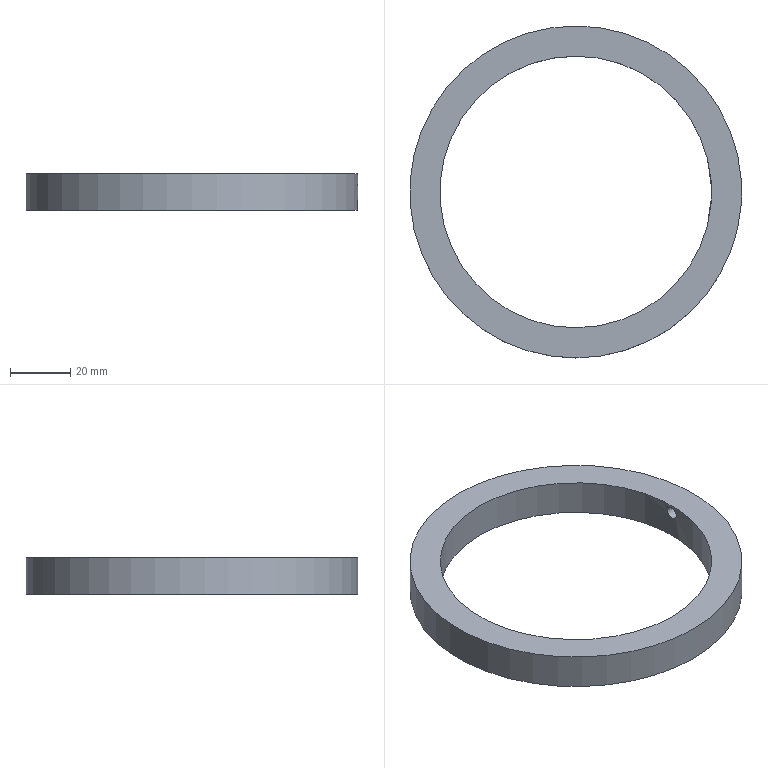Component | NX | CA6140-ZHUZHOU-ZHOUTAO4 | 1 solid | 5 faces | box 110 x 110 x 12 mm | volume 37574 mm3 | cylinder 3 | plane 2 | commonest cylinder face diameters 110 x1 90 x1 4 x1
STEP:
#1=CARTESIAN_POINT('',(0.,0.,0.));
#2=DIRECTION('',(0.,0.,1.));
#3=DIRECTION('',(1.,0.,0.));
#4=AXIS2_PLACEMENT_3D('',#1,#2,#3);
#5=CARTESIAN_POINT('',(0.03562,-45.,-99.951));
#6=VERTEX_POINT('',#5);
#7=CARTESIAN_POINT('',(-0.,-0.,-99.951));
#8=DIRECTION('',(0.,0.,1.));
#9=DIRECTION('',(0.0007915,-1.,0.));
#10=AXIS2_PLACEMENT_3D('',#7,#8,#9);
#11=CIRCLE('',#10,45.);
#12=CARTESIAN_POINT('',(-0.,-0.,-99.951));
#13=DIRECTION('',(0.,0.,-1.));
#14=DIRECTION('',(-0.0007915,1.,0.));
#15=AXIS2_PLACEMENT_3D('',#12,#13,#14);
#16=PLANE('',#15);
#17=CARTESIAN_POINT('',(-45.,0.));
#18=CARTESIAN_POINT('',(-45.,77.942));
#19=CARTESIAN_POINT('',(22.5,38.971));
#20=CARTESIAN_POINT('',(90.,0.));
#21=CARTESIAN_POINT('',(22.5,-38.971));
#22=CARTESIAN_POINT('',(-45.,-77.942));
#23=CARTESIAN_POINT('',(-45.,0.));
#24=(BOUNDED_CURVE()B_SPLINE_CURVE(2,(#17,#18,#19,#20,#21,#22,#23),.UNSPECIFIED.,.T.,.F.)B_SPLINE_CURVE_WITH_KNOTS((1,2,2,2,2,1),(-2.094,0.,2.094,4.189,6.283,8.378),.UNSPECIFIED.)CURVE()GEOMETRIC_REPRESENTATION_ITEM()RATIONAL_B_SPLINE_CURVE((1.,0.5,1.,0.5,1.,0.5,1.))REPRESENTATION_ITEM(''));
#25=(GEOMETRIC_REPRESENTATION_CONTEXT(2)PARAMETRIC_REPRESENTATION_CONTEXT()REPRESENTATION_CONTEXT('',''));
#26=DEFINITIONAL_REPRESENTATION('',(#24),#25);
#27=PCURVE('',#16,#26);
#28=CARTESIAN_POINT('',(-0.,-0.,-99.951));
#29=DIRECTION('',(0.,0.,1.));
#30=DIRECTION('',(0.0007915,-1.,0.));
#31=AXIS2_PLACEMENT_3D('',#28,#29,#30);
#32=CYLINDRICAL_SURFACE('',#31,45.);
#33=CARTESIAN_POINT('',(0.,0.));
#34=DIRECTION('',(1.,0.));
#35=VECTOR('',#34,1.);
#36=LINE('',#33,#35);
#37=(GEOMETRIC_REPRESENTATION_CONTEXT(2)PARAMETRIC_REPRESENTATION_CONTEXT()REPRESENTATION_CONTEXT('',''));
#38=DEFINITIONAL_REPRESENTATION('',(#36),#37);
#39=PCURVE('',#32,#38);
#40=SURFACE_CURVE('',#11,(#27,#39),.PCURVE_S1.);
#41=EDGE_CURVE('',#6,#6,#40,.T.);
#42=ORIENTED_EDGE('',*,*,#41,.T.);
#43=EDGE_LOOP('',(#42));
#44=FACE_BOUND('',#43,.T.);
#45=CARTESIAN_POINT('',(0.04353,-55.,-99.951));
#46=VERTEX_POINT('',#45);
#47=CARTESIAN_POINT('',(-0.04353,55.,-99.951));
#48=VERTEX_POINT('',#47);
#49=CARTESIAN_POINT('',(-0.,-0.,-99.951));
#50=DIRECTION('',(0.,0.,1.));
#51=DIRECTION('',(0.0007915,-1.,0.));
#52=AXIS2_PLACEMENT_3D('',#49,#50,#51);
#53=CIRCLE('',#52,55.);
#54=CARTESIAN_POINT('',(-55.,0.));
#55=CARTESIAN_POINT('',(-55.,95.263));
#56=CARTESIAN_POINT('',(27.5,47.631));
#57=CARTESIAN_POINT('',(110.,0.));
#58=CARTESIAN_POINT('',(27.5,-47.631));
#59=CARTESIAN_POINT('',(-55.,-95.263));
#60=CARTESIAN_POINT('',(-55.,0.));
#61=(BOUNDED_CURVE()B_SPLINE_CURVE(2,(#54,#55,#56,#57,#58,#59,#60),.UNSPECIFIED.,.T.,.F.)B_SPLINE_CURVE_WITH_KNOTS((1,2,2,2,2,1),(-2.094,0.,2.094,4.189,6.283,8.378),.UNSPECIFIED.)CURVE()GEOMETRIC_REPRESENTATION_ITEM()RATIONAL_B_SPLINE_CURVE((1.,0.5,1.,0.5,1.,0.5,1.))REPRESENTATION_ITEM(''));
#62=(GEOMETRIC_REPRESENTATION_CONTEXT(2)PARAMETRIC_REPRESENTATION_CONTEXT()REPRESENTATION_CONTEXT('',''));
#63=DEFINITIONAL_REPRESENTATION('',(#61),#62);
#64=PCURVE('',#16,#63);
#65=CARTESIAN_POINT('',(-0.,-0.,-87.951));
#66=DIRECTION('',(0.,0.,-1.));
#67=DIRECTION('',(-0.0007915,1.,0.));
#68=AXIS2_PLACEMENT_3D('',#65,#66,#67);
#69=CYLINDRICAL_SURFACE('',#68,55.);
#70=CARTESIAN_POINT('',(3.142,12.));
#71=DIRECTION('',(-1.,0.));
#72=VECTOR('',#71,1.);
#73=LINE('',#70,#72);
#74=(GEOMETRIC_REPRESENTATION_CONTEXT(2)PARAMETRIC_REPRESENTATION_CONTEXT()REPRESENTATION_CONTEXT('',''));
#75=DEFINITIONAL_REPRESENTATION('',(#73),#74);
#76=PCURVE('',#69,#75);
#77=SURFACE_CURVE('',#53,(#64,#76),.PCURVE_S1.);
#78=EDGE_CURVE('',#46,#48,#77,.T.);
#79=ORIENTED_EDGE('',*,*,#78,.F.);
#80=CARTESIAN_POINT('',(-0.,-0.,-99.951));
#81=DIRECTION('',(0.,0.,1.));
#82=DIRECTION('',(0.0007915,-1.,0.));
#83=AXIS2_PLACEMENT_3D('',#80,#81,#82);
#84=CIRCLE('',#83,55.);
#85=CARTESIAN_POINT('',(-55.,0.));
#86=CARTESIAN_POINT('',(-55.,95.263));
#87=CARTESIAN_POINT('',(27.5,47.631));
#88=CARTESIAN_POINT('',(110.,0.));
#89=CARTESIAN_POINT('',(27.5,-47.631));
#90=CARTESIAN_POINT('',(-55.,-95.263));
#91=CARTESIAN_POINT('',(-55.,0.));
#92=(BOUNDED_CURVE()B_SPLINE_CURVE(2,(#85,#86,#87,#88,#89,#90,#91),.UNSPECIFIED.,.T.,.F.)B_SPLINE_CURVE_WITH_KNOTS((1,2,2,2,2,1),(-2.094,0.,2.094,4.189,6.283,8.378),.UNSPECIFIED.)CURVE()GEOMETRIC_REPRESENTATION_ITEM()RATIONAL_B_SPLINE_CURVE((1.,0.5,1.,0.5,1.,0.5,1.))REPRESENTATION_ITEM(''));
#93=(GEOMETRIC_REPRESENTATION_CONTEXT(2)PARAMETRIC_REPRESENTATION_CONTEXT()REPRESENTATION_CONTEXT('',''));
#94=DEFINITIONAL_REPRESENTATION('',(#92),#93);
#95=PCURVE('',#16,#94);
#96=CARTESIAN_POINT('',(9.425,12.));
#97=DIRECTION('',(-1.,0.));
#98=VECTOR('',#97,1.);
#99=LINE('',#96,#98);
#100=(GEOMETRIC_REPRESENTATION_CONTEXT(2)PARAMETRIC_REPRESENTATION_CONTEXT()REPRESENTATION_CONTEXT('',''));
#101=DEFINITIONAL_REPRESENTATION('',(#99),#100);
#102=PCURVE('',#69,#101);
#103=SURFACE_CURVE('',#84,(#95,#102),.PCURVE_S1.);
#104=EDGE_CURVE('',#48,#46,#103,.T.);
#105=ORIENTED_EDGE('',*,*,#104,.F.);
#106=EDGE_LOOP('',(#79,#105));
#107=FACE_BOUND('',#106,.T.);
#108=ADVANCED_FACE('',(#44,#107),#16,.T.);
#109=CARTESIAN_POINT('',(0.03562,-45.,-87.951));
#110=VERTEX_POINT('',#109);
#111=CARTESIAN_POINT('',(-0.,-0.,-87.951));
#112=DIRECTION('',(0.,0.,1.));
#113=DIRECTION('',(0.0007915,-1.,0.));
#114=AXIS2_PLACEMENT_3D('',#111,#112,#113);
#115=CIRCLE('',#114,45.);
#116=CARTESIAN_POINT('',(-0.,-0.,-87.951));
#117=DIRECTION('',(0.,0.,1.));
#118=DIRECTION('',(0.0007915,-1.,0.));
#119=AXIS2_PLACEMENT_3D('',#116,#117,#118);
#120=PLANE('',#119);
#121=CARTESIAN_POINT('',(0.,0.));
#122=DIRECTION('',(1.,0.));
#123=AXIS2_PLACEMENT_2D('',#121,#122);
#124=CIRCLE('',#123,45.);
#125=(GEOMETRIC_REPRESENTATION_CONTEXT(2)PARAMETRIC_REPRESENTATION_CONTEXT()REPRESENTATION_CONTEXT('',''));
#126=DEFINITIONAL_REPRESENTATION('',(#124),#125);
#127=PCURVE('',#120,#126);
#128=CARTESIAN_POINT('',(0.,12.));
#129=DIRECTION('',(1.,0.));
#130=VECTOR('',#129,1.);
#131=LINE('',#128,#130);
#132=(GEOMETRIC_REPRESENTATION_CONTEXT(2)PARAMETRIC_REPRESENTATION_CONTEXT()REPRESENTATION_CONTEXT('',''));
#133=DEFINITIONAL_REPRESENTATION('',(#131),#132);
#134=PCURVE('',#32,#133);
#135=SURFACE_CURVE('',#115,(#127,#134),.PCURVE_S1.);
#136=EDGE_CURVE('',#110,#110,#135,.T.);
#137=ORIENTED_EDGE('',*,*,#136,.F.);
#138=EDGE_LOOP('',(#137));
#139=FACE_BOUND('',#138,.T.);
#140=CARTESIAN_POINT('',(-0.04353,55.,-87.951));
#141=VERTEX_POINT('',#140);
#142=CARTESIAN_POINT('',(-0.,-0.,-87.951));
#143=DIRECTION('',(0.,0.,-1.));
#144=DIRECTION('',(-0.0007915,1.,0.));
#145=AXIS2_PLACEMENT_3D('',#142,#143,#144);
#146=CIRCLE('',#145,55.);
#147=CARTESIAN_POINT('',(-55.,0.));
#148=CARTESIAN_POINT('',(-55.,95.263));
#149=CARTESIAN_POINT('',(27.5,47.631));
#150=CARTESIAN_POINT('',(110.,0.));
#151=CARTESIAN_POINT('',(27.5,-47.631));
#152=CARTESIAN_POINT('',(-55.,-95.263));
#153=CARTESIAN_POINT('',(-55.,0.));
#154=(BOUNDED_CURVE()B_SPLINE_CURVE(2,(#147,#148,#149,#150,#151,#152,#153),.UNSPECIFIED.,.T.,.F.)B_SPLINE_CURVE_WITH_KNOTS((1,2,2,2,2,1),(-2.094,0.,2.094,4.189,6.283,8.378),.UNSPECIFIED.)CURVE()GEOMETRIC_REPRESENTATION_ITEM()RATIONAL_B_SPLINE_CURVE((1.,0.5,1.,0.5,1.,0.5,1.))REPRESENTATION_ITEM(''));
#155=(GEOMETRIC_REPRESENTATION_CONTEXT(2)PARAMETRIC_REPRESENTATION_CONTEXT()REPRESENTATION_CONTEXT('',''));
#156=DEFINITIONAL_REPRESENTATION('',(#154),#155);
#157=PCURVE('',#120,#156);
#158=CARTESIAN_POINT('',(0.,0.));
#159=DIRECTION('',(1.,0.));
#160=VECTOR('',#159,1.);
#161=LINE('',#158,#160);
#162=(GEOMETRIC_REPRESENTATION_CONTEXT(2)PARAMETRIC_REPRESENTATION_CONTEXT()REPRESENTATION_CONTEXT('',''));
#163=DEFINITIONAL_REPRESENTATION('',(#161),#162);
#164=PCURVE('',#69,#163);
#165=SURFACE_CURVE('',#146,(#157,#164),.PCURVE_S1.);
#166=EDGE_CURVE('',#141,#141,#165,.T.);
#167=ORIENTED_EDGE('',*,*,#166,.F.);
#168=EDGE_LOOP('',(#167));
#169=FACE_BOUND('',#168,.T.);
#170=ADVANCED_FACE('',(#139,#169),#120,.T.);
#171=ORIENTED_EDGE('',*,*,#78,.T.);
#172=CARTESIAN_POINT('',(-0.04353,55.,-87.951));
#173=CARTESIAN_POINT('',(-0.04353,55.,-99.951));
#174=B_SPLINE_CURVE_WITH_KNOTS('',1,(#172,#173),.UNSPECIFIED.,.F.,.F.,(2,2),(0.,12.),.PIECEWISE_BEZIER_KNOTS.);
#175=CARTESIAN_POINT('',(0.,0.));
#176=DIRECTION('',(0.,1.));
#177=VECTOR('',#176,1.);
#178=LINE('',#175,#177);
#179=(GEOMETRIC_REPRESENTATION_CONTEXT(2)PARAMETRIC_REPRESENTATION_CONTEXT()REPRESENTATION_CONTEXT('',''));
#180=DEFINITIONAL_REPRESENTATION('',(#178),#179);
#181=PCURVE('',#69,#180);
#182=CARTESIAN_POINT('',(6.283,0.));
#183=DIRECTION('',(0.,1.));
#184=VECTOR('',#183,1.);
#185=LINE('',#182,#184);
#186=(GEOMETRIC_REPRESENTATION_CONTEXT(2)PARAMETRIC_REPRESENTATION_CONTEXT()REPRESENTATION_CONTEXT('',''));
#187=DEFINITIONAL_REPRESENTATION('',(#185),#186);
#188=PCURVE('',#69,#187);
#189=SEAM_CURVE('',#174,(#181,#188),.PCURVE_S1.);
#190=EDGE_CURVE('',#141,#48,#189,.T.);
#191=ORIENTED_EDGE('',*,*,#190,.F.);
#192=ORIENTED_EDGE('',*,*,#166,.T.);
#193=ORIENTED_EDGE('',*,*,#190,.T.);
#194=ORIENTED_EDGE('',*,*,#104,.T.);
#195=EDGE_LOOP('',(#171,#191,#192,#193,#194));
#196=FACE_BOUND('',#195,.T.);
#197=CARTESIAN_POINT('',(55.,0.04365,-88.951));
#198=VERTEX_POINT('',#197);
#199=CARTESIAN_POINT('',(55.,0.04365,-88.951));
#200=CARTESIAN_POINT('',(55.,-0.1801,-88.951));
#201=CARTESIAN_POINT('',(54.999,-0.407,-88.989));
#202=CARTESIAN_POINT('',(54.997,-0.6181,-89.063));
#203=CARTESIAN_POINT('',(54.994,-0.8293,-89.137));
#204=CARTESIAN_POINT('',(54.991,-1.031,-89.249));
#205=CARTESIAN_POINT('',(54.987,-1.205,-89.389));
#206=CARTESIAN_POINT('',(54.983,-1.38,-89.528));
#207=CARTESIAN_POINT('',(54.979,-1.533,-89.7));
#208=CARTESIAN_POINT('',(54.975,-1.652,-89.89));
#209=CARTESIAN_POINT('',(54.972,-1.771,-90.08));
#210=CARTESIAN_POINT('',(54.969,-1.858,-90.293));
#211=CARTESIAN_POINT('',(54.967,-1.907,-90.511));
#212=CARTESIAN_POINT('',(54.965,-1.957,-90.729));
#213=CARTESIAN_POINT('',(54.965,-1.969,-90.959));
#214=CARTESIAN_POINT('',(54.966,-1.943,-91.182));
#215=CARTESIAN_POINT('',(54.967,-1.917,-91.404));
#216=CARTESIAN_POINT('',(54.969,-1.853,-91.625));
#217=CARTESIAN_POINT('',(54.972,-1.755,-91.826));
#218=CARTESIAN_POINT('',(54.975,-1.657,-92.027));
#219=CARTESIAN_POINT('',(54.979,-1.523,-92.214));
#220=CARTESIAN_POINT('',(54.983,-1.364,-92.371));
#221=CARTESIAN_POINT('',(54.987,-1.205,-92.529));
#222=CARTESIAN_POINT('',(54.991,-1.017,-92.661));
#223=CARTESIAN_POINT('',(54.994,-0.8143,-92.757));
#224=CARTESIAN_POINT('',(54.997,-0.612,-92.853));
#225=CARTESIAN_POINT('',(54.999,-0.3904,-92.916));
#226=CARTESIAN_POINT('',(55.,-0.1678,-92.939));
#227=CARTESIAN_POINT('',(55.,0.05473,-92.963));
#228=CARTESIAN_POINT('',(55.,0.2844,-92.949));
#229=CARTESIAN_POINT('',(54.998,0.5022,-92.897));
#230=CARTESIAN_POINT('',(54.996,0.7199,-92.846));
#231=CARTESIAN_POINT('',(54.992,0.9318,-92.757));
#232=CARTESIAN_POINT('',(54.989,1.12,-92.636));
#233=CARTESIAN_POINT('',(54.985,1.309,-92.516));
#234=CARTESIAN_POINT('',(54.98,1.479,-92.361));
#235=CARTESIAN_POINT('',(54.976,1.617,-92.185));
#236=CARTESIAN_POINT('',(54.972,1.756,-92.009));
#237=CARTESIAN_POINT('',(54.968,1.865,-91.806));
#238=CARTESIAN_POINT('',(54.966,1.937,-91.594));
#239=CARTESIAN_POINT('',(54.963,2.009,-91.382));
#240=CARTESIAN_POINT('',(54.962,2.046,-91.155));
#241=CARTESIAN_POINT('',(54.962,2.044,-90.931));
#242=CARTESIAN_POINT('',(54.962,2.041,-90.707));
#243=CARTESIAN_POINT('',(54.964,2.001,-90.481));
#244=CARTESIAN_POINT('',(54.966,1.924,-90.271));
#245=CARTESIAN_POINT('',(54.969,1.848,-90.06));
#246=CARTESIAN_POINT('',(54.973,1.735,-89.86));
#247=CARTESIAN_POINT('',(54.977,1.594,-89.687));
#248=CARTESIAN_POINT('',(54.981,1.452,-89.513));
#249=CARTESIAN_POINT('',(54.985,1.279,-89.362));
#250=CARTESIAN_POINT('',(54.989,1.088,-89.245));
#251=CARTESIAN_POINT('',(54.993,0.8971,-89.128));
#252=CARTESIAN_POINT('',(54.996,0.6833,-89.043));
#253=CARTESIAN_POINT('',(54.998,0.4644,-88.995));
#254=CARTESIAN_POINT('',(54.999,0.3265,-88.966));
#255=CARTESIAN_POINT('',(55.,0.1847,-88.951));
#256=CARTESIAN_POINT('',(55.,0.04365,-88.951));
#257=B_SPLINE_CURVE_WITH_KNOTS('',3,(#199,#200,#201,#202,#203,#204,#205,#206,#207,#208,#209,#210,#211,#212,#213,#214,#215,#216,#217,#218,#219,#220,#221,#222,#223,#224,#225,#226,#227,#228,#229,#230,#231,#232,#233,#234,#235,#236,#237,#238,#239,#240,#241,#242,#243,#244,#245,#246,#247,#248,#249,#250,#251,#252,#253,#254,#255,#256),.UNSPECIFIED.,.T.,.F.,(1,3,3,3,3,3,3,3,3,3,3,3,3,3,3,3,3,3,3,3,3,1),(-0.03354,0.,0.05368,0.1074,0.1611,0.2148,0.2685,0.3221,0.3758,0.4295,0.4832,0.5369,0.5906,0.6443,0.698,0.7517,0.8054,0.859,0.9127,0.9665,1.,1.054),.UNSPECIFIED.);
#258=CARTESIAN_POINT('',(1.571,0.9999));
#259=CARTESIAN_POINT('',(1.572,0.9999));
#260=CARTESIAN_POINT('',(1.573,1.003));
#261=CARTESIAN_POINT('',(1.576,1.019));
#262=CARTESIAN_POINT('',(1.579,1.044));
#263=CARTESIAN_POINT('',(1.581,1.079));
#264=CARTESIAN_POINT('',(1.584,1.124));
#265=CARTESIAN_POINT('',(1.586,1.179));
#266=CARTESIAN_POINT('',(1.588,1.243));
#267=CARTESIAN_POINT('',(1.59,1.316));
#268=CARTESIAN_POINT('',(1.593,1.398));
#269=CARTESIAN_POINT('',(1.595,1.487));
#270=CARTESIAN_POINT('',(1.597,1.584));
#271=CARTESIAN_POINT('',(1.598,1.689));
#272=CARTESIAN_POINT('',(1.6,1.8));
#273=CARTESIAN_POINT('',(1.601,1.917));
#274=CARTESIAN_POINT('',(1.603,2.04));
#275=CARTESIAN_POINT('',(1.604,2.168));
#276=CARTESIAN_POINT('',(1.605,2.3));
#277=CARTESIAN_POINT('',(1.606,2.436));
#278=CARTESIAN_POINT('',(1.606,2.574));
#279=CARTESIAN_POINT('',(1.607,2.714));
#280=CARTESIAN_POINT('',(1.607,2.856));
#281=CARTESIAN_POINT('',(1.607,3.));
#282=CARTESIAN_POINT('',(1.607,3.142));
#283=CARTESIAN_POINT('',(1.607,3.284));
#284=CARTESIAN_POINT('',(1.606,3.424));
#285=CARTESIAN_POINT('',(1.606,3.563));
#286=CARTESIAN_POINT('',(1.605,3.699));
#287=CARTESIAN_POINT('',(1.604,3.831));
#288=CARTESIAN_POINT('',(1.603,3.958));
#289=CARTESIAN_POINT('',(1.601,4.081));
#290=CARTESIAN_POINT('',(1.6,4.199));
#291=CARTESIAN_POINT('',(1.598,4.31));
#292=CARTESIAN_POINT('',(1.597,4.415));
#293=CARTESIAN_POINT('',(1.595,4.512));
#294=CARTESIAN_POINT('',(1.593,4.602));
#295=CARTESIAN_POINT('',(1.59,4.683));
#296=CARTESIAN_POINT('',(1.588,4.756));
#297=CARTESIAN_POINT('',(1.586,4.82));
#298=CARTESIAN_POINT('',(1.584,4.875));
#299=CARTESIAN_POINT('',(1.581,4.92));
#300=CARTESIAN_POINT('',(1.579,4.956));
#301=CARTESIAN_POINT('',(1.576,4.981));
#302=CARTESIAN_POINT('',(1.573,4.996));
#303=CARTESIAN_POINT('',(1.571,5.001));
#304=CARTESIAN_POINT('',(1.568,4.996));
#305=CARTESIAN_POINT('',(1.566,4.981));
#306=CARTESIAN_POINT('',(1.563,4.956));
#307=CARTESIAN_POINT('',(1.561,4.921));
#308=CARTESIAN_POINT('',(1.558,4.876));
#309=CARTESIAN_POINT('',(1.556,4.821));
#310=CARTESIAN_POINT('',(1.553,4.757));
#311=CARTESIAN_POINT('',(1.551,4.685));
#312=CARTESIAN_POINT('',(1.549,4.603));
#313=CARTESIAN_POINT('',(1.547,4.514));
#314=CARTESIAN_POINT('',(1.545,4.416));
#315=CARTESIAN_POINT('',(1.543,4.312));
#316=CARTESIAN_POINT('',(1.542,4.201));
#317=CARTESIAN_POINT('',(1.54,4.084));
#318=CARTESIAN_POINT('',(1.539,3.961));
#319=CARTESIAN_POINT('',(1.538,3.833));
#320=CARTESIAN_POINT('',(1.537,3.701));
#321=CARTESIAN_POINT('',(1.536,3.566));
#322=CARTESIAN_POINT('',(1.535,3.427));
#323=CARTESIAN_POINT('',(1.535,3.286));
#324=CARTESIAN_POINT('',(1.534,3.144));
#325=CARTESIAN_POINT('',(1.534,3.002));
#326=CARTESIAN_POINT('',(1.534,2.859));
#327=CARTESIAN_POINT('',(1.535,2.717));
#328=CARTESIAN_POINT('',(1.535,2.576));
#329=CARTESIAN_POINT('',(1.536,2.437));
#330=CARTESIAN_POINT('',(1.537,2.302));
#331=CARTESIAN_POINT('',(1.538,2.171));
#332=CARTESIAN_POINT('',(1.539,2.043));
#333=CARTESIAN_POINT('',(1.54,1.919));
#334=CARTESIAN_POINT('',(1.542,1.802));
#335=CARTESIAN_POINT('',(1.543,1.691));
#336=CARTESIAN_POINT('',(1.545,1.586));
#337=CARTESIAN_POINT('',(1.547,1.489));
#338=CARTESIAN_POINT('',(1.549,1.399));
#339=CARTESIAN_POINT('',(1.551,1.317));
#340=CARTESIAN_POINT('',(1.553,1.244));
#341=CARTESIAN_POINT('',(1.556,1.18));
#342=CARTESIAN_POINT('',(1.558,1.125));
#343=CARTESIAN_POINT('',(1.561,1.08));
#344=CARTESIAN_POINT('',(1.563,1.044));
#345=CARTESIAN_POINT('',(1.566,1.019));
#346=CARTESIAN_POINT('',(1.568,1.003));
#347=CARTESIAN_POINT('',(1.57,0.9999));
#348=CARTESIAN_POINT('',(1.571,0.9999));
#349=B_SPLINE_CURVE_WITH_KNOTS('',3,(#258,#259,#260,#261,#262,#263,#264,#265,#266,#267,#268,#269,#270,#271,#272,#273,#274,#275,#276,#277,#278,#279,#280,#281,#282,#283,#284,#285,#286,#287,#288,#289,#290,#291,#292,#293,#294,#295,#296,#297,#298,#299,#300,#301,#302,#303,#304,#305,#306,#307,#308,#309,#310,#311,#312,#313,#314,#315,#316,#317,#318,#319,#320,#321,#322,#323,#324,#325,#326,#327,#328,#329,#330,#331,#332,#333,#334,#335,#336,#337,#338,#339,#340,#341,#342,#343,#344,#345,#346,#347,#348),.UNSPECIFIED.,.T.,.F.,(4,1,1,1,1,1,1,1,1,1,1,1,1,1,1,1,1,1,1,1,1,1,1,1,1,1,1,1,1,1,1,1,1,1,1,1,1,1,1,1,1,1,1,1,1,1,1,1,1,1,1,1,1,1,1,1,1,1,1,1,1,1,1,1,1,1,1,1,1,1,1,1,1,1,1,1,1,1,1,1,1,1,1,1,1,1,1,1,4),(0.,0.01136,0.02273,0.03409,0.04545,0.05682,0.06818,0.07955,0.09091,0.1023,0.1136,0.125,0.1364,0.1477,0.1591,0.1705,0.1818,0.1932,0.2045,0.2159,0.2273,0.2386,0.25,0.2614,0.2727,0.2841,0.2955,0.3068,0.3182,0.3295,0.3409,0.3523,0.3636,0.375,0.3864,0.3977,0.4091,0.4205,0.4318,0.4432,0.4545,0.4659,0.4773,0.4886,0.5,0.5114,0.5227,0.5341,0.5455,0.5568,0.5682,0.5795,0.5909,0.6023,0.6136,0.625,0.6364,0.6477,0.6591,0.6705,0.6818,0.6932,0.7045,0.7159,0.7273,0.7386,0.75,0.7614,0.7727,0.7841,0.7955,0.8068,0.8182,0.8295,0.8409,0.8523,0.8636,0.875,0.8864,0.8977,0.9091,0.9205,0.9318,0.9432,0.9545,0.9659,0.9773,0.9886,1.),.QUASI_UNIFORM_KNOTS.);
#350=(GEOMETRIC_REPRESENTATION_CONTEXT(2)PARAMETRIC_REPRESENTATION_CONTEXT()REPRESENTATION_CONTEXT('',''));
#351=DEFINITIONAL_REPRESENTATION('',(#349),#350);
#352=PCURVE('',#69,#351);
#353=CARTESIAN_POINT('',(60.,0.04761,-90.951));
#354=DIRECTION('',(-1.,-0.0007915,0.));
#355=DIRECTION('',(0.,0.,1.));
#356=AXIS2_PLACEMENT_3D('',#353,#354,#355);
#357=CYLINDRICAL_SURFACE('',#356,2.);
#358=CARTESIAN_POINT('',(6.283,5.));
#359=CARTESIAN_POINT('',(0.,5.));
#360=B_SPLINE_CURVE_WITH_KNOTS('',1,(#358,#359),.UNSPECIFIED.,.F.,.F.,(2,2),(0.,1.),.PIECEWISE_BEZIER_KNOTS.);
#361=(GEOMETRIC_REPRESENTATION_CONTEXT(2)PARAMETRIC_REPRESENTATION_CONTEXT()REPRESENTATION_CONTEXT('',''));
#362=DEFINITIONAL_REPRESENTATION('',(#360),#361);
#363=PCURVE('',#357,#362);
#364=SURFACE_CURVE('',#257,(#352,#363),.PCURVE_S1.);
#365=EDGE_CURVE('',#198,#198,#364,.T.);
#366=ORIENTED_EDGE('',*,*,#365,.F.);
#367=EDGE_LOOP('',(#366));
#368=FACE_BOUND('',#367,.T.);
#369=ADVANCED_FACE('',(#196,#368),#69,.T.);
#370=ORIENTED_EDGE('',*,*,#136,.F.);
#371=CARTESIAN_POINT('',(0.03562,-45.,-99.951));
#372=CARTESIAN_POINT('',(0.03562,-45.,-87.951));
#373=B_SPLINE_CURVE_WITH_KNOTS('',1,(#371,#372),.UNSPECIFIED.,.F.,.F.,(2,2),(0.,12.),.PIECEWISE_BEZIER_KNOTS.);
#374=CARTESIAN_POINT('',(0.,0.));
#375=DIRECTION('',(0.,1.));
#376=VECTOR('',#375,1.);
#377=LINE('',#374,#376);
#378=(GEOMETRIC_REPRESENTATION_CONTEXT(2)PARAMETRIC_REPRESENTATION_CONTEXT()REPRESENTATION_CONTEXT('',''));
#379=DEFINITIONAL_REPRESENTATION('',(#377),#378);
#380=PCURVE('',#32,#379);
#381=CARTESIAN_POINT('',(6.283,0.));
#382=DIRECTION('',(0.,1.));
#383=VECTOR('',#382,1.);
#384=LINE('',#381,#383);
#385=(GEOMETRIC_REPRESENTATION_CONTEXT(2)PARAMETRIC_REPRESENTATION_CONTEXT()REPRESENTATION_CONTEXT('',''));
#386=DEFINITIONAL_REPRESENTATION('',(#384),#385);
#387=PCURVE('',#32,#386);
#388=SEAM_CURVE('',#373,(#380,#387),.PCURVE_S1.);
#389=EDGE_CURVE('',#6,#110,#388,.T.);
#390=ORIENTED_EDGE('',*,*,#389,.F.);
#391=ORIENTED_EDGE('',*,*,#41,.T.);
#392=ORIENTED_EDGE('',*,*,#389,.T.);
#393=EDGE_LOOP('',(#370,#390,#391,#392));
#394=FACE_BOUND('',#393,.F.);
#395=CARTESIAN_POINT('',(45.,0.03574,-88.951));
#396=VERTEX_POINT('',#395);
#397=CARTESIAN_POINT('',(45.,0.03574,-88.951));
#398=CARTESIAN_POINT('',(45.,-0.188,-88.951));
#399=CARTESIAN_POINT('',(44.999,-0.4148,-88.989));
#400=CARTESIAN_POINT('',(44.996,-0.6259,-89.063));
#401=CARTESIAN_POINT('',(44.993,-0.837,-89.137));
#402=CARTESIAN_POINT('',(44.988,-1.038,-89.249));
#403=CARTESIAN_POINT('',(44.984,-1.213,-89.388));
#404=CARTESIAN_POINT('',(44.979,-1.388,-89.528));
#405=CARTESIAN_POINT('',(44.974,-1.541,-89.7));
#406=CARTESIAN_POINT('',(44.969,-1.66,-89.89));
#407=CARTESIAN_POINT('',(44.965,-1.778,-90.079));
#408=CARTESIAN_POINT('',(44.961,-1.866,-90.292));
#409=CARTESIAN_POINT('',(44.959,-1.915,-90.511));
#410=CARTESIAN_POINT('',(44.957,-1.965,-90.729));
#411=CARTESIAN_POINT('',(44.957,-1.977,-90.959));
#412=CARTESIAN_POINT('',(44.958,-1.951,-91.181));
#413=CARTESIAN_POINT('',(44.959,-1.925,-91.403));
#414=CARTESIAN_POINT('',(44.962,-1.861,-91.624));
#415=CARTESIAN_POINT('',(44.965,-1.763,-91.825));
#416=CARTESIAN_POINT('',(44.969,-1.665,-92.026));
#417=CARTESIAN_POINT('',(44.974,-1.531,-92.213));
#418=CARTESIAN_POINT('',(44.979,-1.372,-92.371));
#419=CARTESIAN_POINT('',(44.984,-1.213,-92.529));
#420=CARTESIAN_POINT('',(44.989,-1.025,-92.661));
#421=CARTESIAN_POINT('',(44.992,-0.8228,-92.757));
#422=CARTESIAN_POINT('',(44.996,-0.6206,-92.853));
#423=CARTESIAN_POINT('',(44.999,-0.399,-92.916));
#424=CARTESIAN_POINT('',(45.,-0.1763,-92.939));
#425=CARTESIAN_POINT('',(45.001,0.04613,-92.963));
#426=CARTESIAN_POINT('',(45.,0.2758,-92.949));
#427=CARTESIAN_POINT('',(44.997,0.4935,-92.898));
#428=CARTESIAN_POINT('',(44.995,0.7112,-92.846));
#429=CARTESIAN_POINT('',(44.991,0.9231,-92.757));
#430=CARTESIAN_POINT('',(44.986,1.112,-92.637));
#431=CARTESIAN_POINT('',(44.982,1.3,-92.516));
#432=CARTESIAN_POINT('',(44.976,1.471,-92.362));
#433=CARTESIAN_POINT('',(44.971,1.609,-92.186));
#434=CARTESIAN_POINT('',(44.966,1.747,-92.01));
#435=CARTESIAN_POINT('',(44.962,1.857,-91.807));
#436=CARTESIAN_POINT('',(44.959,1.929,-91.595));
#437=CARTESIAN_POINT('',(44.956,2.001,-91.383));
#438=CARTESIAN_POINT('',(44.954,2.038,-91.156));
#439=CARTESIAN_POINT('',(44.954,2.036,-90.932));
#440=CARTESIAN_POINT('',(44.954,2.034,-90.709));
#441=CARTESIAN_POINT('',(44.956,1.993,-90.482));
#442=CARTESIAN_POINT('',(44.959,1.917,-90.272));
#443=CARTESIAN_POINT('',(44.962,1.841,-90.061));
#444=CARTESIAN_POINT('',(44.967,1.728,-89.861));
#445=CARTESIAN_POINT('',(44.972,1.587,-89.688));
#446=CARTESIAN_POINT('',(44.977,1.445,-89.514));
#447=CARTESIAN_POINT('',(44.982,1.272,-89.363));
#448=CARTESIAN_POINT('',(44.987,1.081,-89.246));
#449=CARTESIAN_POINT('',(44.992,0.8905,-89.129));
#450=CARTESIAN_POINT('',(44.995,0.6767,-89.043));
#451=CARTESIAN_POINT('',(44.998,0.4578,-88.996));
#452=CARTESIAN_POINT('',(44.999,0.3195,-88.966));
#453=CARTESIAN_POINT('',(45.,0.1772,-88.951));
#454=CARTESIAN_POINT('',(45.,0.03574,-88.951));
#455=B_SPLINE_CURVE_WITH_KNOTS('',3,(#397,#398,#399,#400,#401,#402,#403,#404,#405,#406,#407,#408,#409,#410,#411,#412,#413,#414,#415,#416,#417,#418,#419,#420,#421,#422,#423,#424,#425,#426,#427,#428,#429,#430,#431,#432,#433,#434,#435,#436,#437,#438,#439,#440,#441,#442,#443,#444,#445,#446,#447,#448,#449,#450,#451,#452,#453,#454),.UNSPECIFIED.,.T.,.F.,(1,3,3,3,3,3,3,3,3,3,3,3,3,3,3,3,3,3,3,3,3,1),(-0.03365,0.,0.05367,0.1073,0.161,0.2148,0.2684,0.3221,0.3758,0.4295,0.4832,0.5369,0.5905,0.6442,0.6979,0.7516,0.8053,0.8589,0.9126,0.9663,1.,1.054),.UNSPECIFIED.);
#456=CARTESIAN_POINT('',(1.571,11.));
#457=CARTESIAN_POINT('',(1.57,11.));
#458=CARTESIAN_POINT('',(1.568,10.997));
#459=CARTESIAN_POINT('',(1.564,10.981));
#460=CARTESIAN_POINT('',(1.561,10.956));
#461=CARTESIAN_POINT('',(1.558,10.921));
#462=CARTESIAN_POINT('',(1.555,10.876));
#463=CARTESIAN_POINT('',(1.552,10.821));
#464=CARTESIAN_POINT('',(1.549,10.757));
#465=CARTESIAN_POINT('',(1.547,10.684));
#466=CARTESIAN_POINT('',(1.544,10.602));
#467=CARTESIAN_POINT('',(1.542,10.513));
#468=CARTESIAN_POINT('',(1.539,10.416));
#469=CARTESIAN_POINT('',(1.537,10.311));
#470=CARTESIAN_POINT('',(1.535,10.2));
#471=CARTESIAN_POINT('',(1.533,10.083));
#472=CARTESIAN_POINT('',(1.532,9.96));
#473=CARTESIAN_POINT('',(1.53,9.832));
#474=CARTESIAN_POINT('',(1.529,9.7));
#475=CARTESIAN_POINT('',(1.528,9.564));
#476=CARTESIAN_POINT('',(1.527,9.426));
#477=CARTESIAN_POINT('',(1.527,9.286));
#478=CARTESIAN_POINT('',(1.526,9.144));
#479=CARTESIAN_POINT('',(1.526,9.));
#480=CARTESIAN_POINT('',(1.526,8.857));
#481=CARTESIAN_POINT('',(1.527,8.716));
#482=CARTESIAN_POINT('',(1.527,8.576));
#483=CARTESIAN_POINT('',(1.528,8.437));
#484=CARTESIAN_POINT('',(1.529,8.301));
#485=CARTESIAN_POINT('',(1.53,8.169));
#486=CARTESIAN_POINT('',(1.532,8.042));
#487=CARTESIAN_POINT('',(1.533,7.919));
#488=CARTESIAN_POINT('',(1.535,7.801));
#489=CARTESIAN_POINT('',(1.537,7.69));
#490=CARTESIAN_POINT('',(1.539,7.585));
#491=CARTESIAN_POINT('',(1.542,7.488));
#492=CARTESIAN_POINT('',(1.544,7.398));
#493=CARTESIAN_POINT('',(1.547,7.317));
#494=CARTESIAN_POINT('',(1.549,7.244));
#495=CARTESIAN_POINT('',(1.552,7.18));
#496=CARTESIAN_POINT('',(1.555,7.125));
#497=CARTESIAN_POINT('',(1.558,7.08));
#498=CARTESIAN_POINT('',(1.561,7.044));
#499=CARTESIAN_POINT('',(1.564,7.019));
#500=CARTESIAN_POINT('',(1.568,7.004));
#501=CARTESIAN_POINT('',(1.571,6.999));
#502=CARTESIAN_POINT('',(1.574,7.004));
#503=CARTESIAN_POINT('',(1.577,7.019));
#504=CARTESIAN_POINT('',(1.58,7.044));
#505=CARTESIAN_POINT('',(1.583,7.079));
#506=CARTESIAN_POINT('',(1.586,7.124));
#507=CARTESIAN_POINT('',(1.589,7.179));
#508=CARTESIAN_POINT('',(1.592,7.243));
#509=CARTESIAN_POINT('',(1.595,7.315));
#510=CARTESIAN_POINT('',(1.597,7.397));
#511=CARTESIAN_POINT('',(1.6,7.486));
#512=CARTESIAN_POINT('',(1.602,7.584));
#513=CARTESIAN_POINT('',(1.604,7.688));
#514=CARTESIAN_POINT('',(1.606,7.799));
#515=CARTESIAN_POINT('',(1.608,7.916));
#516=CARTESIAN_POINT('',(1.61,8.039));
#517=CARTESIAN_POINT('',(1.611,8.167));
#518=CARTESIAN_POINT('',(1.612,8.299));
#519=CARTESIAN_POINT('',(1.613,8.434));
#520=CARTESIAN_POINT('',(1.614,8.573));
#521=CARTESIAN_POINT('',(1.615,8.714));
#522=CARTESIAN_POINT('',(1.615,8.856));
#523=CARTESIAN_POINT('',(1.615,8.998));
#524=CARTESIAN_POINT('',(1.615,9.141));
#525=CARTESIAN_POINT('',(1.615,9.283));
#526=CARTESIAN_POINT('',(1.614,9.424));
#527=CARTESIAN_POINT('',(1.613,9.563));
#528=CARTESIAN_POINT('',(1.613,9.698));
#529=CARTESIAN_POINT('',(1.611,9.829));
#530=CARTESIAN_POINT('',(1.61,9.957));
#531=CARTESIAN_POINT('',(1.608,10.081));
#532=CARTESIAN_POINT('',(1.606,10.198));
#533=CARTESIAN_POINT('',(1.604,10.309));
#534=CARTESIAN_POINT('',(1.602,10.414));
#535=CARTESIAN_POINT('',(1.6,10.511));
#536=CARTESIAN_POINT('',(1.597,10.601));
#537=CARTESIAN_POINT('',(1.595,10.683));
#538=CARTESIAN_POINT('',(1.592,10.756));
#539=CARTESIAN_POINT('',(1.589,10.82));
#540=CARTESIAN_POINT('',(1.586,10.875));
#541=CARTESIAN_POINT('',(1.583,10.92));
#542=CARTESIAN_POINT('',(1.58,10.955));
#543=CARTESIAN_POINT('',(1.577,10.981));
#544=CARTESIAN_POINT('',(1.574,10.997));
#545=CARTESIAN_POINT('',(1.572,11.));
#546=CARTESIAN_POINT('',(1.571,11.));
#547=B_SPLINE_CURVE_WITH_KNOTS('',3,(#456,#457,#458,#459,#460,#461,#462,#463,#464,#465,#466,#467,#468,#469,#470,#471,#472,#473,#474,#475,#476,#477,#478,#479,#480,#481,#482,#483,#484,#485,#486,#487,#488,#489,#490,#491,#492,#493,#494,#495,#496,#497,#498,#499,#500,#501,#502,#503,#504,#505,#506,#507,#508,#509,#510,#511,#512,#513,#514,#515,#516,#517,#518,#519,#520,#521,#522,#523,#524,#525,#526,#527,#528,#529,#530,#531,#532,#533,#534,#535,#536,#537,#538,#539,#540,#541,#542,#543,#544,#545,#546),.UNSPECIFIED.,.T.,.F.,(4,1,1,1,1,1,1,1,1,1,1,1,1,1,1,1,1,1,1,1,1,1,1,1,1,1,1,1,1,1,1,1,1,1,1,1,1,1,1,1,1,1,1,1,1,1,1,1,1,1,1,1,1,1,1,1,1,1,1,1,1,1,1,1,1,1,1,1,1,1,1,1,1,1,1,1,1,1,1,1,1,1,1,1,1,1,1,1,4),(0.,0.01136,0.02273,0.03409,0.04545,0.05682,0.06818,0.07955,0.09091,0.1023,0.1136,0.125,0.1364,0.1477,0.1591,0.1705,0.1818,0.1932,0.2045,0.2159,0.2273,0.2386,0.25,0.2614,0.2727,0.2841,0.2955,0.3068,0.3182,0.3295,0.3409,0.3523,0.3636,0.375,0.3864,0.3977,0.4091,0.4205,0.4318,0.4432,0.4545,0.4659,0.4773,0.4886,0.5,0.5114,0.5227,0.5341,0.5455,0.5568,0.5682,0.5795,0.5909,0.6023,0.6136,0.625,0.6364,0.6477,0.6591,0.6705,0.6818,0.6932,0.7045,0.7159,0.7273,0.7386,0.75,0.7614,0.7727,0.7841,0.7955,0.8068,0.8182,0.8295,0.8409,0.8523,0.8636,0.875,0.8864,0.8977,0.9091,0.9205,0.9318,0.9432,0.9545,0.9659,0.9773,0.9886,1.),.QUASI_UNIFORM_KNOTS.);
#548=(GEOMETRIC_REPRESENTATION_CONTEXT(2)PARAMETRIC_REPRESENTATION_CONTEXT()REPRESENTATION_CONTEXT('',''));
#549=DEFINITIONAL_REPRESENTATION('',(#547),#548);
#550=PCURVE('',#32,#549);
#551=CARTESIAN_POINT('',(6.283,15.));
#552=CARTESIAN_POINT('',(0.,15.));
#553=B_SPLINE_CURVE_WITH_KNOTS('',1,(#551,#552),.UNSPECIFIED.,.F.,.F.,(2,2),(0.,1.),.PIECEWISE_BEZIER_KNOTS.);
#554=(GEOMETRIC_REPRESENTATION_CONTEXT(2)PARAMETRIC_REPRESENTATION_CONTEXT()REPRESENTATION_CONTEXT('',''));
#555=DEFINITIONAL_REPRESENTATION('',(#553),#554);
#556=PCURVE('',#357,#555);
#557=SURFACE_CURVE('',#455,(#550,#556),.PCURVE_S1.);
#558=EDGE_CURVE('',#396,#396,#557,.T.);
#559=ORIENTED_EDGE('',*,*,#558,.F.);
#560=EDGE_LOOP('',(#559));
#561=FACE_BOUND('',#560,.F.);
#562=ADVANCED_FACE('',(#394,#561),#32,.F.);
#563=ORIENTED_EDGE('',*,*,#365,.F.);
#564=CARTESIAN_POINT('',(55.,0.04365,-88.951));
#565=CARTESIAN_POINT('',(45.,0.03574,-88.951));
#566=B_SPLINE_CURVE_WITH_KNOTS('',1,(#564,#565),.UNSPECIFIED.,.F.,.F.,(2,2),(5.,15.),.PIECEWISE_BEZIER_KNOTS.);
#567=CARTESIAN_POINT('',(6.283,0.));
#568=DIRECTION('',(0.,1.));
#569=VECTOR('',#568,1.);
#570=LINE('',#567,#569);
#571=(GEOMETRIC_REPRESENTATION_CONTEXT(2)PARAMETRIC_REPRESENTATION_CONTEXT()REPRESENTATION_CONTEXT('',''));
#572=DEFINITIONAL_REPRESENTATION('',(#570),#571);
#573=PCURVE('',#357,#572);
#574=CARTESIAN_POINT('',(0.,0.));
#575=DIRECTION('',(0.,1.));
#576=VECTOR('',#575,1.);
#577=LINE('',#574,#576);
#578=(GEOMETRIC_REPRESENTATION_CONTEXT(2)PARAMETRIC_REPRESENTATION_CONTEXT()REPRESENTATION_CONTEXT('',''));
#579=DEFINITIONAL_REPRESENTATION('',(#577),#578);
#580=PCURVE('',#357,#579);
#581=SEAM_CURVE('',#566,(#573,#580),.PCURVE_S1.);
#582=EDGE_CURVE('',#198,#396,#581,.T.);
#583=ORIENTED_EDGE('',*,*,#582,.T.);
#584=ORIENTED_EDGE('',*,*,#558,.T.);
#585=ORIENTED_EDGE('',*,*,#582,.F.);
#586=EDGE_LOOP('',(#563,#583,#584,#585));
#587=FACE_BOUND('',#586,.F.);
#588=ADVANCED_FACE('',(#587),#357,.F.);
#589=CLOSED_SHELL('',(#108,#170,#369,#562,#588));
#590=MANIFOLD_SOLID_BREP('',#589);
#591=(LENGTH_UNIT()NAMED_UNIT(*)SI_UNIT(.MILLI.,.METRE.));
#592=UNCERTAINTY_MEASURE_WITH_UNIT(LENGTH_MEASURE(0.01),#591,'','');
#593=(NAMED_UNIT(*)PLANE_ANGLE_UNIT()SI_UNIT($,.RADIAN.));
#594=(NAMED_UNIT(*)SI_UNIT($,.STERADIAN.)SOLID_ANGLE_UNIT());
#595=(GEOMETRIC_REPRESENTATION_CONTEXT(3)GLOBAL_UNCERTAINTY_ASSIGNED_CONTEXT((#592))GLOBAL_UNIT_ASSIGNED_CONTEXT((#591,#593,#594))REPRESENTATION_CONTEXT('',''));
#596=ADVANCED_BREP_SHAPE_REPRESENTATION('',(#4,#590),#595);